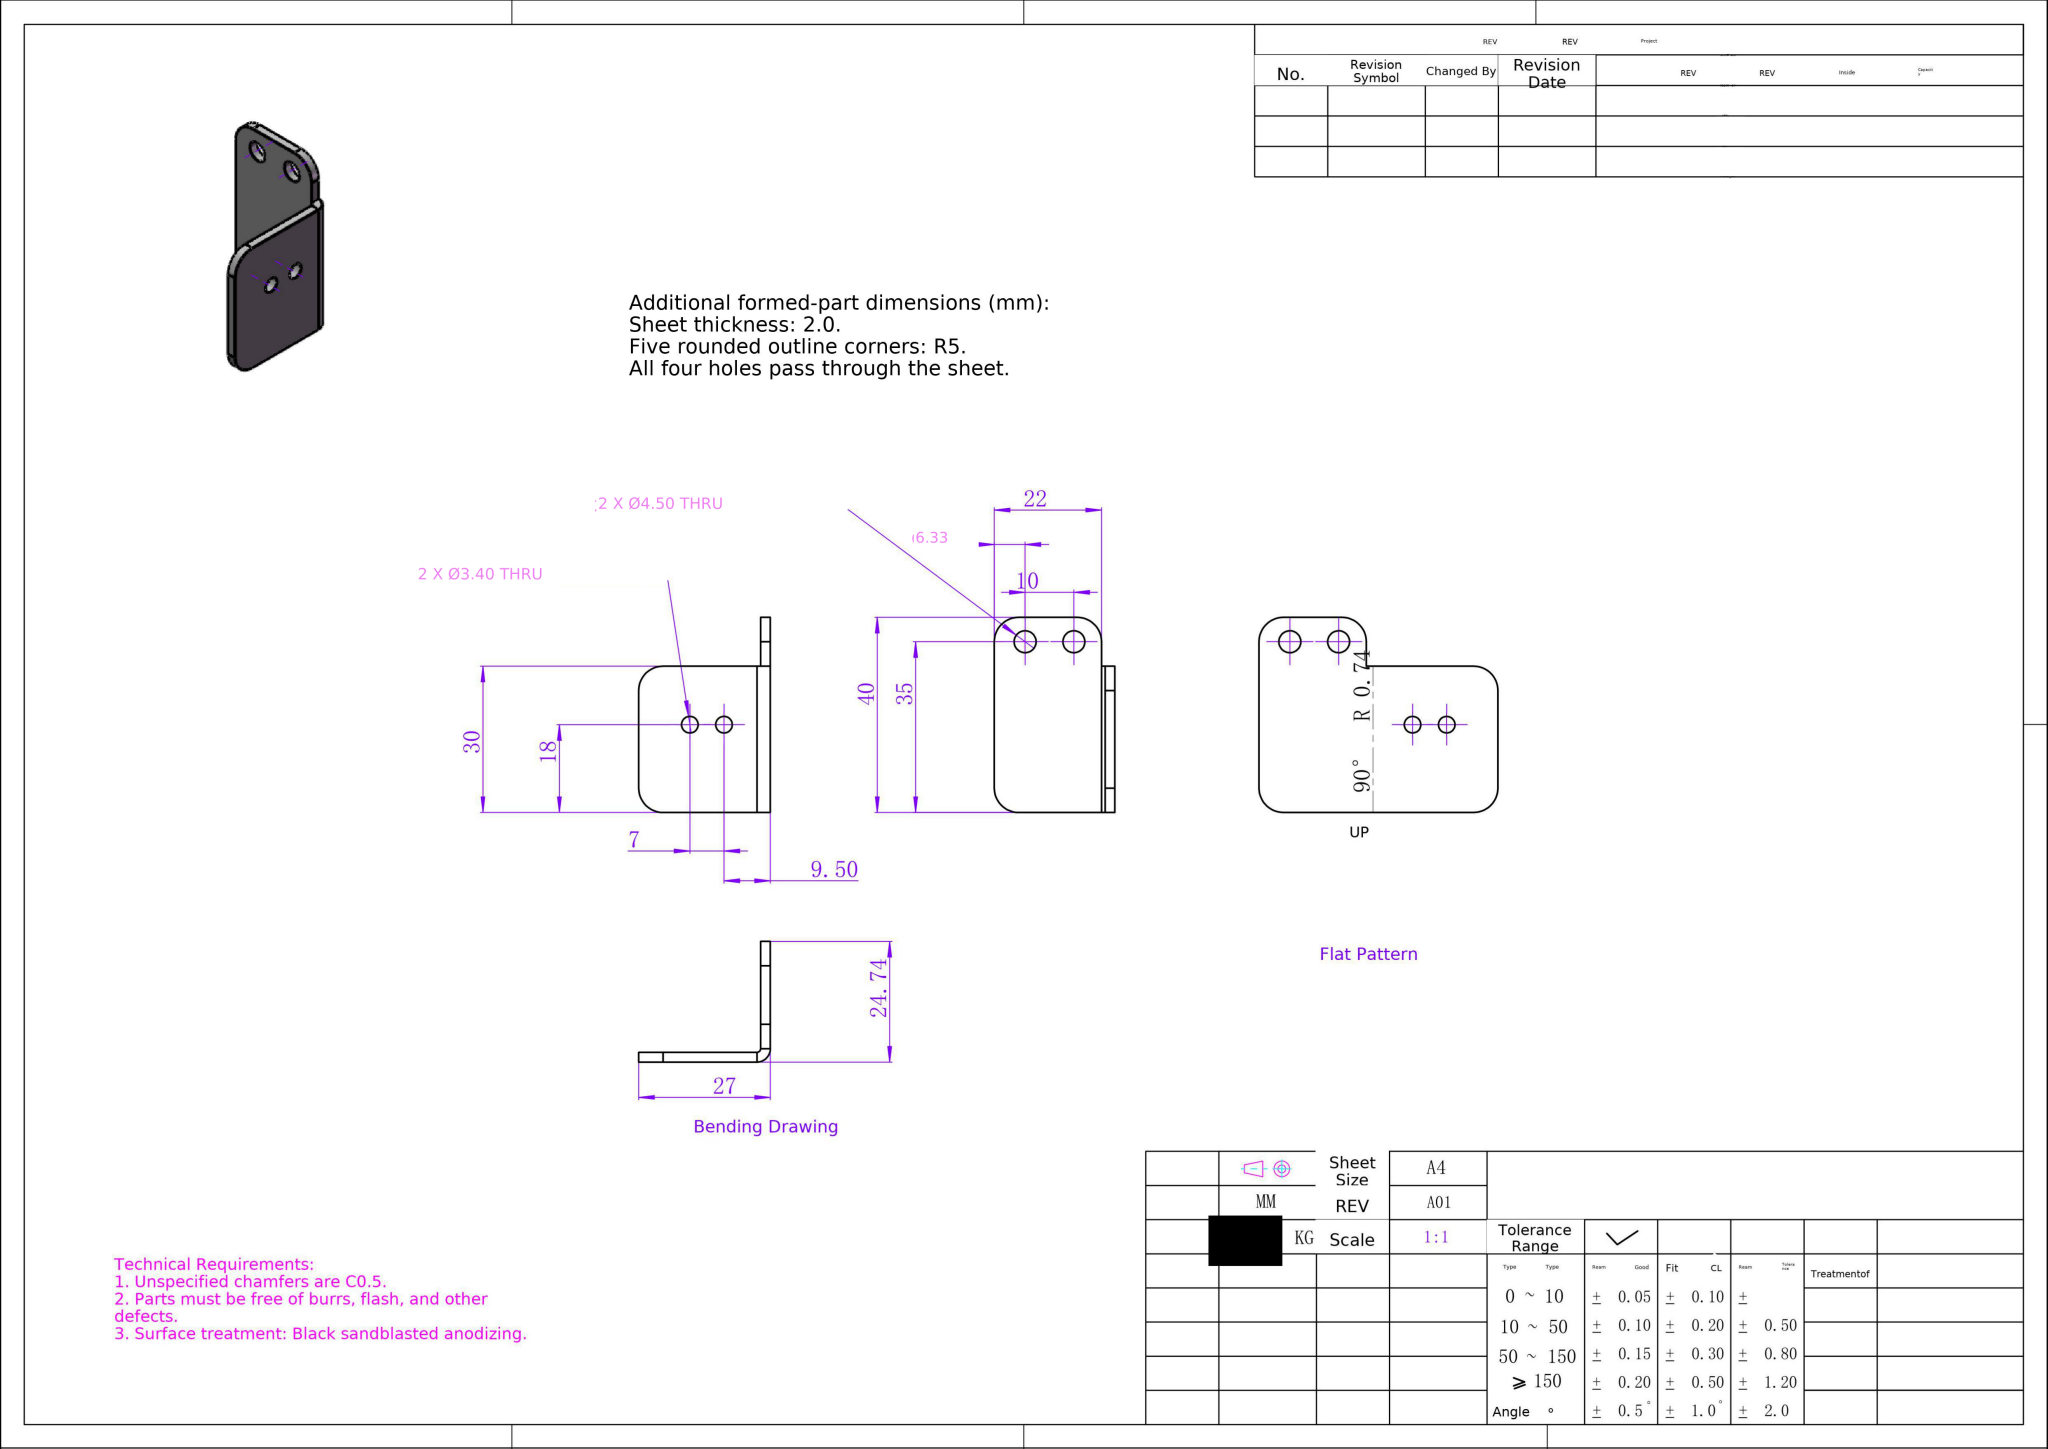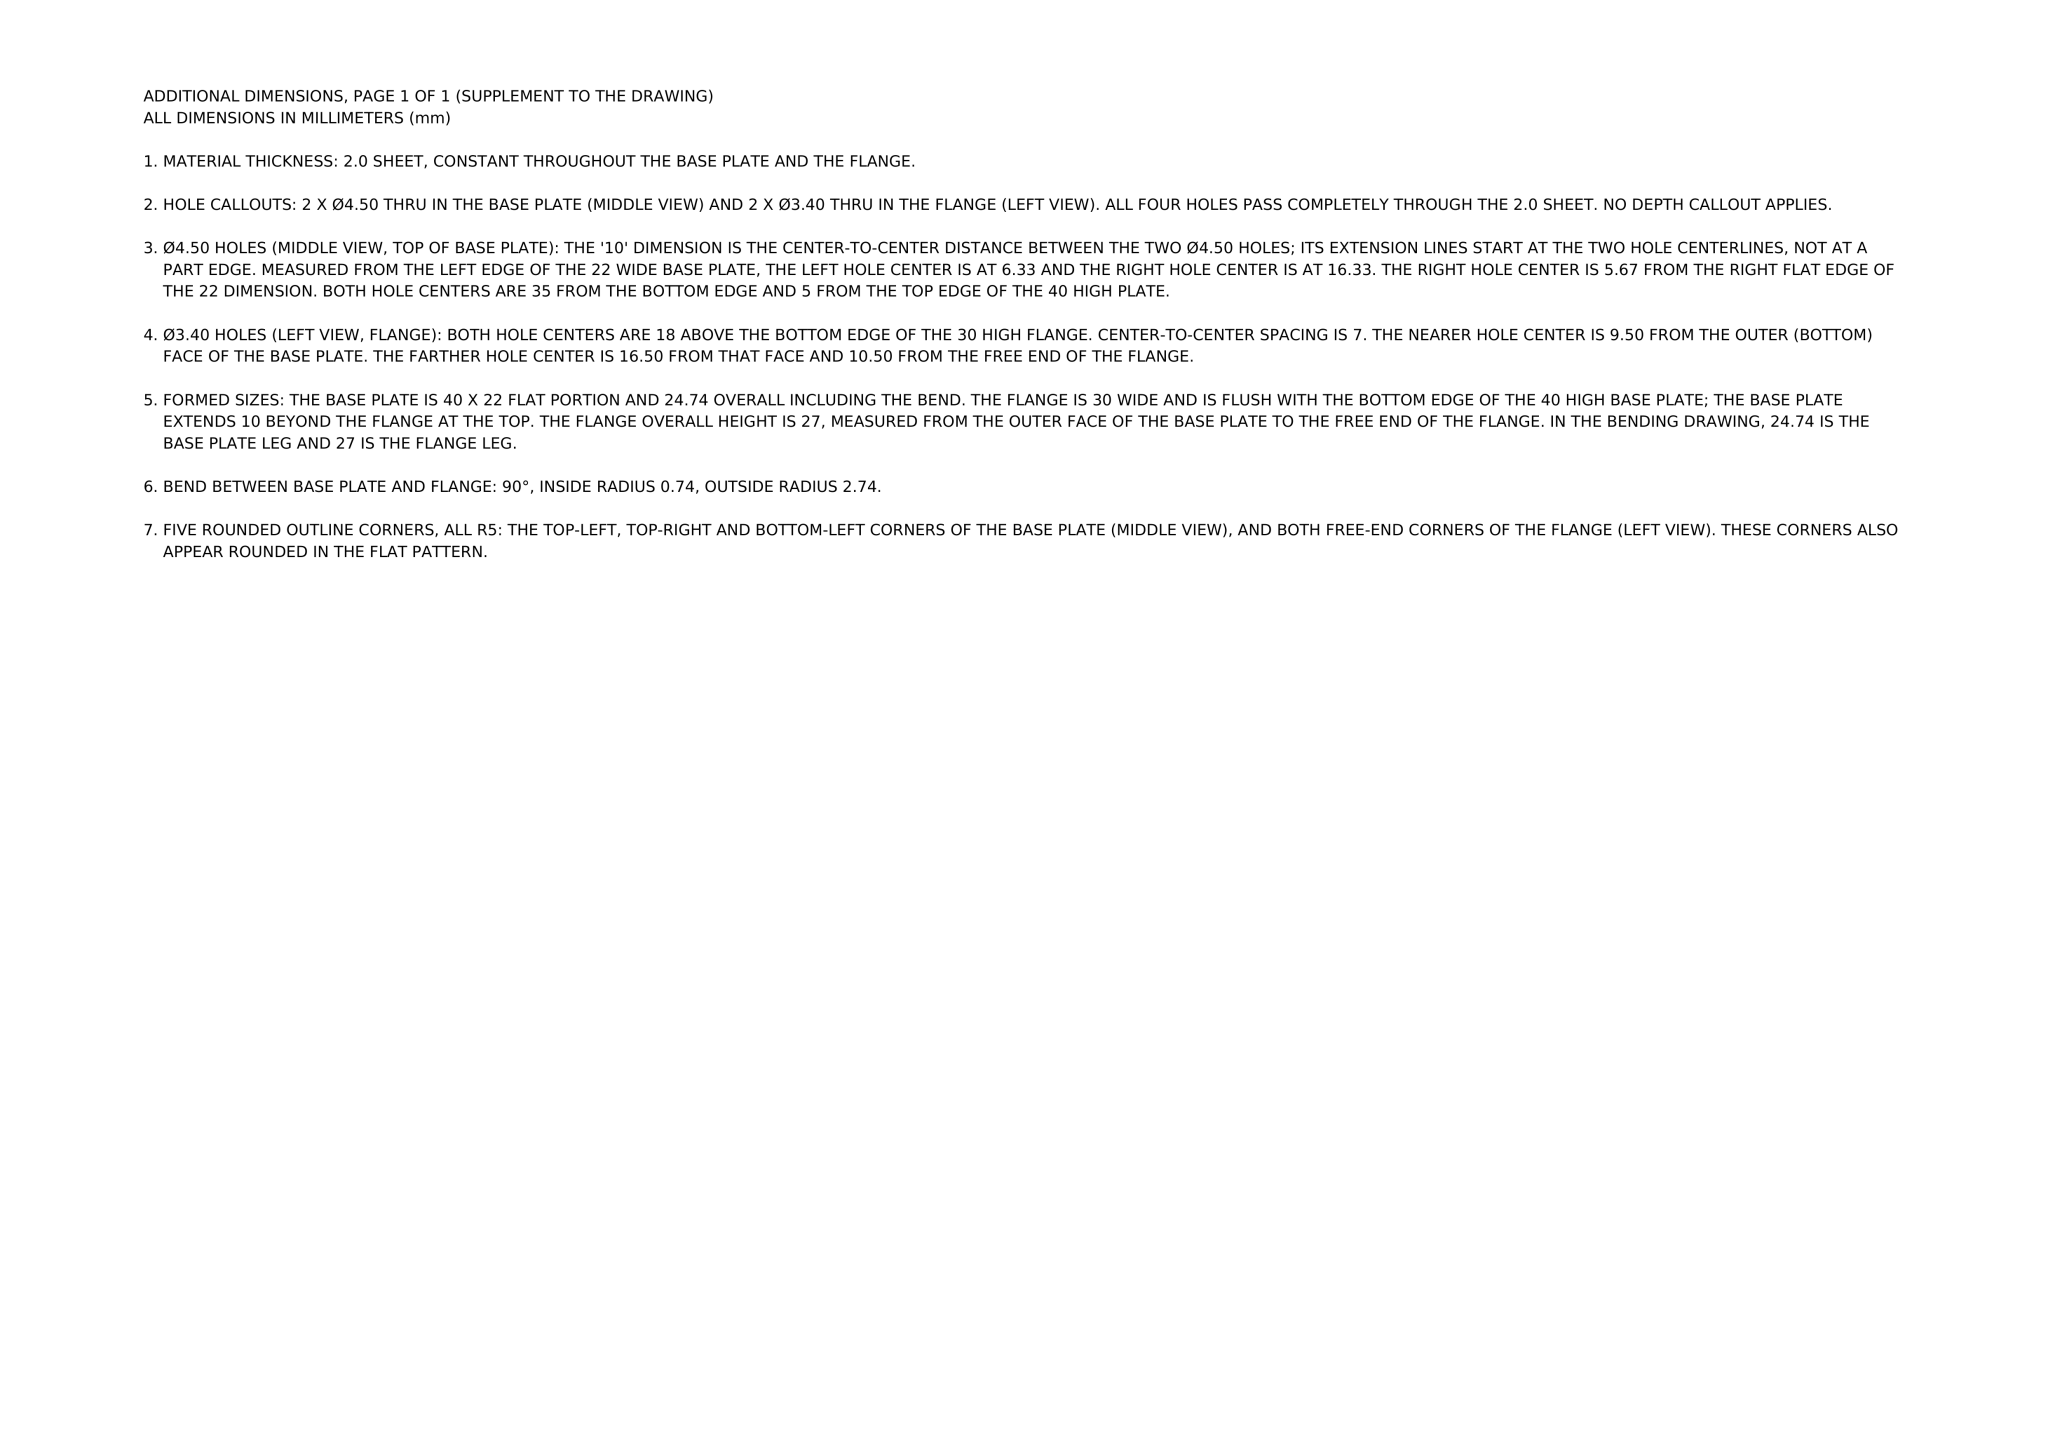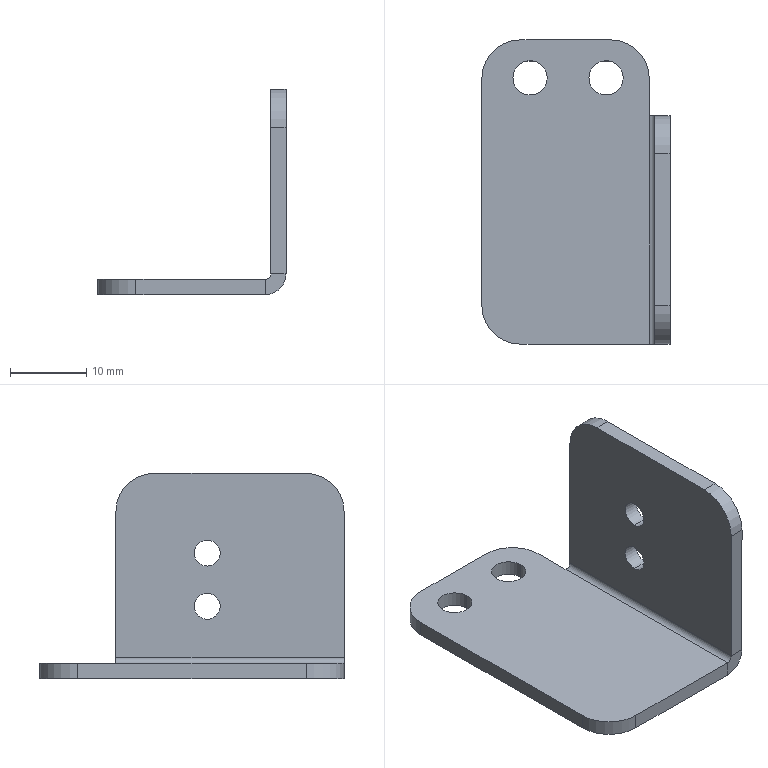Part | NX | mm | 1 solid | 28 faces | box 24.74 x 40 x 27 mm | volume 3226 mm3 | cylinder 15 | plane 13 | commonest cylinder face diameters 10 x5 3.4 x4 4.5 x4 5.473 x1 1.473 x1
STEP:
#1=COLOUR_RGB('',0.6471,0.6471,0.6471);
#2=FILL_AREA_STYLE_COLOUR('',#1);
#3=FILL_AREA_STYLE('',(#2));
#4=SURFACE_STYLE_FILL_AREA(#3);
#5=SURFACE_SIDE_STYLE('',(#4));
#6=SURFACE_STYLE_USAGE(.BOTH.,#5);
#7=PRESENTATION_STYLE_ASSIGNMENT((#6));
#8=CARTESIAN_POINT('',(46.729,-192.154,16.2));
#9=VERTEX_POINT('',#8);
#10=CARTESIAN_POINT('',(46.729,-192.154,12.8));
#11=VERTEX_POINT('',#10);
#12=CARTESIAN_POINT('',(46.729,-192.154,14.5));
#13=DIRECTION('',(1.,0.,-0.));
#14=DIRECTION('',(-0.,0.,-1.));
#15=AXIS2_PLACEMENT_3D('',#12,#13,#14);
#16=CIRCLE('',#15,1.7);
#17=EDGE_CURVE('',#9,#11,#16,.T.);
#18=ORIENTED_EDGE('',*,*,#17,.F.);
#19=CARTESIAN_POINT('',(48.729,-192.154,16.2));
#20=VERTEX_POINT('',#19);
#21=CARTESIAN_POINT('',(48.729,-192.154,16.2));
#22=DIRECTION('',(1.,0.,-0.));
#23=VECTOR('',#22,1000.);
#24=LINE('',#21,#23);
#25=EDGE_CURVE('',#9,#20,#24,.T.);
#26=ORIENTED_EDGE('',*,*,#25,.T.);
#27=CARTESIAN_POINT('',(48.729,-192.154,12.8));
#28=VERTEX_POINT('',#27);
#29=CARTESIAN_POINT('',(48.729,-192.154,14.5));
#30=DIRECTION('',(1.,0.,-0.));
#31=DIRECTION('',(-0.,0.,-1.));
#32=AXIS2_PLACEMENT_3D('',#29,#30,#31);
#33=CIRCLE('',#32,1.7);
#34=EDGE_CURVE('',#20,#28,#33,.T.);
#35=ORIENTED_EDGE('',*,*,#34,.T.);
#36=CARTESIAN_POINT('',(48.729,-192.154,12.8));
#37=DIRECTION('',(1.,0.,-0.));
#38=VECTOR('',#37,1000.);
#39=LINE('',#36,#38);
#40=EDGE_CURVE('',#11,#28,#39,.T.);
#41=ORIENTED_EDGE('',*,*,#40,.F.);
#42=EDGE_LOOP('',(#18,#26,#35,#41));
#43=FACE_OUTER_BOUND('',#42,.T.);
#44=CARTESIAN_POINT('',(48.729,-192.154,14.5));
#45=DIRECTION('',(1.,0.,-0.));
#46=DIRECTION('',(-0.,0.,-1.));
#47=AXIS2_PLACEMENT_3D('',#44,#45,#46);
#48=CYLINDRICAL_SURFACE('',#47,1.7);
#49=ADVANCED_FACE('',(#43),#48,.F.);
#50=CARTESIAN_POINT('',(46.729,-192.154,9.2));
#51=VERTEX_POINT('',#50);
#52=CARTESIAN_POINT('',(46.729,-192.154,5.8));
#53=VERTEX_POINT('',#52);
#54=CARTESIAN_POINT('',(46.729,-192.154,7.5));
#55=DIRECTION('',(1.,0.,-0.));
#56=DIRECTION('',(-0.,0.,-1.));
#57=AXIS2_PLACEMENT_3D('',#54,#55,#56);
#58=CIRCLE('',#57,1.7);
#59=EDGE_CURVE('',#51,#53,#58,.T.);
#60=ORIENTED_EDGE('',*,*,#59,.F.);
#61=CARTESIAN_POINT('',(48.729,-192.154,9.2));
#62=VERTEX_POINT('',#61);
#63=CARTESIAN_POINT('',(48.729,-192.154,9.2));
#64=DIRECTION('',(1.,0.,-0.));
#65=VECTOR('',#64,1000.);
#66=LINE('',#63,#65);
#67=EDGE_CURVE('',#51,#62,#66,.T.);
#68=ORIENTED_EDGE('',*,*,#67,.T.);
#69=CARTESIAN_POINT('',(48.729,-192.154,5.8));
#70=VERTEX_POINT('',#69);
#71=CARTESIAN_POINT('',(48.729,-192.154,7.5));
#72=DIRECTION('',(1.,0.,-0.));
#73=DIRECTION('',(-0.,0.,-1.));
#74=AXIS2_PLACEMENT_3D('',#71,#72,#73);
#75=CIRCLE('',#74,1.7);
#76=EDGE_CURVE('',#62,#70,#75,.T.);
#77=ORIENTED_EDGE('',*,*,#76,.T.);
#78=CARTESIAN_POINT('',(48.729,-192.154,5.8));
#79=DIRECTION('',(1.,0.,-0.));
#80=VECTOR('',#79,1000.);
#81=LINE('',#78,#80);
#82=EDGE_CURVE('',#53,#70,#81,.T.);
#83=ORIENTED_EDGE('',*,*,#82,.F.);
#84=EDGE_LOOP('',(#60,#68,#77,#83));
#85=FACE_OUTER_BOUND('',#84,.T.);
#86=CARTESIAN_POINT('',(48.729,-192.154,7.5));
#87=DIRECTION('',(1.,0.,-0.));
#88=DIRECTION('',(-0.,0.,-1.));
#89=AXIS2_PLACEMENT_3D('',#86,#87,#88);
#90=CYLINDRICAL_SURFACE('',#89,1.7);
#91=ADVANCED_FACE('',(#85),#90,.F.);
#92=CARTESIAN_POINT('',(38.067,-175.154,-2.));
#93=VERTEX_POINT('',#92);
#94=CARTESIAN_POINT('',(42.567,-175.154,-2.));
#95=VERTEX_POINT('',#94);
#96=CARTESIAN_POINT('',(40.317,-175.154,-2.));
#97=DIRECTION('',(0.,0.,1.));
#98=DIRECTION('',(1.,0.,0.));
#99=AXIS2_PLACEMENT_3D('',#96,#97,#98);
#100=CIRCLE('',#99,2.25);
#101=EDGE_CURVE('',#93,#95,#100,.T.);
#102=ORIENTED_EDGE('',*,*,#101,.F.);
#103=CARTESIAN_POINT('',(38.067,-175.154,0.));
#104=VERTEX_POINT('',#103);
#105=CARTESIAN_POINT('',(38.067,-175.154,0.));
#106=DIRECTION('',(0.,0.,1.));
#107=VECTOR('',#106,1000.);
#108=LINE('',#105,#107);
#109=EDGE_CURVE('',#93,#104,#108,.T.);
#110=ORIENTED_EDGE('',*,*,#109,.T.);
#111=CARTESIAN_POINT('',(42.567,-175.154,0.));
#112=VERTEX_POINT('',#111);
#113=CARTESIAN_POINT('',(40.317,-175.154,0.));
#114=DIRECTION('',(0.,0.,1.));
#115=DIRECTION('',(1.,0.,0.));
#116=AXIS2_PLACEMENT_3D('',#113,#114,#115);
#117=CIRCLE('',#116,2.25);
#118=EDGE_CURVE('',#104,#112,#117,.T.);
#119=ORIENTED_EDGE('',*,*,#118,.T.);
#120=CARTESIAN_POINT('',(42.567,-175.154,0.));
#121=DIRECTION('',(0.,0.,1.));
#122=VECTOR('',#121,1000.);
#123=LINE('',#120,#122);
#124=EDGE_CURVE('',#95,#112,#123,.T.);
#125=ORIENTED_EDGE('',*,*,#124,.F.);
#126=EDGE_LOOP('',(#102,#110,#119,#125));
#127=FACE_OUTER_BOUND('',#126,.T.);
#128=CARTESIAN_POINT('',(40.317,-175.154,0.));
#129=DIRECTION('',(0.,0.,1.));
#130=DIRECTION('',(1.,0.,0.));
#131=AXIS2_PLACEMENT_3D('',#128,#129,#130);
#132=CYLINDRICAL_SURFACE('',#131,2.25);
#133=ADVANCED_FACE('',(#127),#132,.F.);
#134=CARTESIAN_POINT('',(28.067,-175.154,-2.));
#135=VERTEX_POINT('',#134);
#136=CARTESIAN_POINT('',(32.567,-175.154,-2.));
#137=VERTEX_POINT('',#136);
#138=CARTESIAN_POINT('',(30.317,-175.154,-2.));
#139=DIRECTION('',(0.,0.,1.));
#140=DIRECTION('',(1.,0.,0.));
#141=AXIS2_PLACEMENT_3D('',#138,#139,#140);
#142=CIRCLE('',#141,2.25);
#143=EDGE_CURVE('',#135,#137,#142,.T.);
#144=ORIENTED_EDGE('',*,*,#143,.F.);
#145=CARTESIAN_POINT('',(28.067,-175.154,0.));
#146=VERTEX_POINT('',#145);
#147=CARTESIAN_POINT('',(28.067,-175.154,0.));
#148=DIRECTION('',(0.,0.,1.));
#149=VECTOR('',#148,1000.);
#150=LINE('',#147,#149);
#151=EDGE_CURVE('',#135,#146,#150,.T.);
#152=ORIENTED_EDGE('',*,*,#151,.T.);
#153=CARTESIAN_POINT('',(32.567,-175.154,0.));
#154=VERTEX_POINT('',#153);
#155=CARTESIAN_POINT('',(30.317,-175.154,0.));
#156=DIRECTION('',(0.,0.,1.));
#157=DIRECTION('',(1.,0.,0.));
#158=AXIS2_PLACEMENT_3D('',#155,#156,#157);
#159=CIRCLE('',#158,2.25);
#160=EDGE_CURVE('',#146,#154,#159,.T.);
#161=ORIENTED_EDGE('',*,*,#160,.T.);
#162=CARTESIAN_POINT('',(32.567,-175.154,0.));
#163=DIRECTION('',(0.,0.,1.));
#164=VECTOR('',#163,1000.);
#165=LINE('',#162,#164);
#166=EDGE_CURVE('',#137,#154,#165,.T.);
#167=ORIENTED_EDGE('',*,*,#166,.F.);
#168=EDGE_LOOP('',(#144,#152,#161,#167));
#169=FACE_OUTER_BOUND('',#168,.T.);
#170=CARTESIAN_POINT('',(30.317,-175.154,0.));
#171=DIRECTION('',(0.,0.,1.));
#172=DIRECTION('',(1.,0.,0.));
#173=AXIS2_PLACEMENT_3D('',#170,#171,#172);
#174=CYLINDRICAL_SURFACE('',#173,2.25);
#175=ADVANCED_FACE('',(#169),#174,.F.);
#176=CARTESIAN_POINT('',(45.993,-180.154,-2.));
#177=VERTEX_POINT('',#176);
#178=CARTESIAN_POINT('',(45.993,-175.154,-2.));
#179=VERTEX_POINT('',#178);
#180=CARTESIAN_POINT('',(45.993,-170.154,-2.));
#181=DIRECTION('',(-0.,1.,0.));
#182=VECTOR('',#181,1000.);
#183=LINE('',#180,#182);
#184=EDGE_CURVE('',#177,#179,#183,.T.);
#185=ORIENTED_EDGE('',*,*,#184,.T.);
#186=CARTESIAN_POINT('',(45.993,-175.154,0.));
#187=VERTEX_POINT('',#186);
#188=CARTESIAN_POINT('',(45.993,-175.154,-2.));
#189=DIRECTION('',(0.,0.,1.));
#190=VECTOR('',#189,1000.);
#191=LINE('',#188,#190);
#192=EDGE_CURVE('',#179,#187,#191,.T.);
#193=ORIENTED_EDGE('',*,*,#192,.T.);
#194=CARTESIAN_POINT('',(45.993,-180.154,0.));
#195=VERTEX_POINT('',#194);
#196=CARTESIAN_POINT('',(45.993,-170.154,0.));
#197=DIRECTION('',(-0.,1.,0.));
#198=VECTOR('',#197,1000.);
#199=LINE('',#196,#198);
#200=EDGE_CURVE('',#195,#187,#199,.T.);
#201=ORIENTED_EDGE('',*,*,#200,.F.);
#202=CARTESIAN_POINT('',(45.993,-180.154,0.));
#203=DIRECTION('',(0.,0.,-1.));
#204=VECTOR('',#203,1000.);
#205=LINE('',#202,#204);
#206=EDGE_CURVE('',#195,#177,#205,.T.);
#207=ORIENTED_EDGE('',*,*,#206,.T.);
#208=EDGE_LOOP('',(#185,#193,#201,#207));
#209=FACE_OUTER_BOUND('',#208,.T.);
#210=CARTESIAN_POINT('',(45.993,-170.154,-2.));
#211=DIRECTION('',(1.,0.,0.));
#212=DIRECTION('',(-0.,1.,0.));
#213=AXIS2_PLACEMENT_3D('',#210,#211,#212);
#214=PLANE('',#213);
#215=ADVANCED_FACE('',(#209),#214,.T.);
#216=CARTESIAN_POINT('',(23.993,-175.154,0.));
#217=VERTEX_POINT('',#216);
#218=CARTESIAN_POINT('',(23.993,-205.154,0.));
#219=VERTEX_POINT('',#218);
#220=CARTESIAN_POINT('',(23.993,-170.154,0.));
#221=DIRECTION('',(0.,-1.,0.));
#222=VECTOR('',#221,1000.);
#223=LINE('',#220,#222);
#224=EDGE_CURVE('',#217,#219,#223,.T.);
#225=ORIENTED_EDGE('',*,*,#224,.F.);
#226=CARTESIAN_POINT('',(23.993,-175.154,-2.));
#227=VERTEX_POINT('',#226);
#228=CARTESIAN_POINT('',(23.993,-175.154,-2.));
#229=DIRECTION('',(0.,0.,-1.));
#230=VECTOR('',#229,1000.);
#231=LINE('',#228,#230);
#232=EDGE_CURVE('',#217,#227,#231,.T.);
#233=ORIENTED_EDGE('',*,*,#232,.T.);
#234=CARTESIAN_POINT('',(23.993,-205.154,-2.));
#235=VERTEX_POINT('',#234);
#236=CARTESIAN_POINT('',(23.993,-170.154,-2.));
#237=DIRECTION('',(0.,-1.,0.));
#238=VECTOR('',#237,1000.);
#239=LINE('',#236,#238);
#240=EDGE_CURVE('',#227,#235,#239,.T.);
#241=ORIENTED_EDGE('',*,*,#240,.T.);
#242=CARTESIAN_POINT('',(23.993,-205.154,-2.));
#243=DIRECTION('',(0.,0.,1.));
#244=VECTOR('',#243,1000.);
#245=LINE('',#242,#244);
#246=EDGE_CURVE('',#235,#219,#245,.T.);
#247=ORIENTED_EDGE('',*,*,#246,.T.);
#248=EDGE_LOOP('',(#225,#233,#241,#247));
#249=FACE_OUTER_BOUND('',#248,.T.);
#250=CARTESIAN_POINT('',(23.993,-170.154,-2.));
#251=DIRECTION('',(-1.,-0.,0.));
#252=DIRECTION('',(0.,-1.,0.));
#253=AXIS2_PLACEMENT_3D('',#250,#251,#252);
#254=PLANE('',#253);
#255=ADVANCED_FACE('',(#249),#254,.T.);
#256=CARTESIAN_POINT('',(40.993,-170.154,-2.));
#257=VERTEX_POINT('',#256);
#258=CARTESIAN_POINT('',(28.993,-170.154,-2.));
#259=VERTEX_POINT('',#258);
#260=CARTESIAN_POINT('',(23.993,-170.154,-2.));
#261=DIRECTION('',(-1.,0.,0.));
#262=VECTOR('',#261,1000.);
#263=LINE('',#260,#262);
#264=EDGE_CURVE('',#257,#259,#263,.T.);
#265=ORIENTED_EDGE('',*,*,#264,.T.);
#266=CARTESIAN_POINT('',(28.993,-170.154,0.));
#267=VERTEX_POINT('',#266);
#268=CARTESIAN_POINT('',(28.993,-170.154,-2.));
#269=DIRECTION('',(0.,0.,1.));
#270=VECTOR('',#269,1000.);
#271=LINE('',#268,#270);
#272=EDGE_CURVE('',#259,#267,#271,.T.);
#273=ORIENTED_EDGE('',*,*,#272,.T.);
#274=CARTESIAN_POINT('',(40.993,-170.154,0.));
#275=VERTEX_POINT('',#274);
#276=CARTESIAN_POINT('',(23.993,-170.154,0.));
#277=DIRECTION('',(-1.,0.,0.));
#278=VECTOR('',#277,1000.);
#279=LINE('',#276,#278);
#280=EDGE_CURVE('',#275,#267,#279,.T.);
#281=ORIENTED_EDGE('',*,*,#280,.F.);
#282=CARTESIAN_POINT('',(40.993,-170.154,-2.));
#283=DIRECTION('',(0.,0.,-1.));
#284=VECTOR('',#283,1000.);
#285=LINE('',#282,#284);
#286=EDGE_CURVE('',#275,#257,#285,.T.);
#287=ORIENTED_EDGE('',*,*,#286,.T.);
#288=EDGE_LOOP('',(#265,#273,#281,#287));
#289=FACE_OUTER_BOUND('',#288,.T.);
#290=CARTESIAN_POINT('',(23.993,-170.154,-2.));
#291=DIRECTION('',(0.,1.,0.));
#292=DIRECTION('',(0.,0.,1.));
#293=AXIS2_PLACEMENT_3D('',#290,#291,#292);
#294=PLANE('',#293);
#295=ADVANCED_FACE('',(#289),#294,.T.);
#296=CARTESIAN_POINT('',(28.993,-210.154,0.));
#297=VERTEX_POINT('',#296);
#298=CARTESIAN_POINT('',(45.993,-210.154,0.));
#299=VERTEX_POINT('',#298);
#300=CARTESIAN_POINT('',(23.993,-210.154,0.));
#301=DIRECTION('',(1.,0.,0.));
#302=VECTOR('',#301,1000.);
#303=LINE('',#300,#302);
#304=EDGE_CURVE('',#297,#299,#303,.T.);
#305=ORIENTED_EDGE('',*,*,#304,.F.);
#306=CARTESIAN_POINT('',(28.993,-210.154,-2.));
#307=VERTEX_POINT('',#306);
#308=CARTESIAN_POINT('',(28.993,-210.154,-2.));
#309=DIRECTION('',(0.,0.,-1.));
#310=VECTOR('',#309,1000.);
#311=LINE('',#308,#310);
#312=EDGE_CURVE('',#297,#307,#311,.T.);
#313=ORIENTED_EDGE('',*,*,#312,.T.);
#314=CARTESIAN_POINT('',(45.993,-210.154,-2.));
#315=VERTEX_POINT('',#314);
#316=CARTESIAN_POINT('',(23.993,-210.154,-2.));
#317=DIRECTION('',(1.,0.,0.));
#318=VECTOR('',#317,1000.);
#319=LINE('',#316,#318);
#320=EDGE_CURVE('',#307,#315,#319,.T.);
#321=ORIENTED_EDGE('',*,*,#320,.T.);
#322=CARTESIAN_POINT('',(45.993,-210.154,-2.));
#323=DIRECTION('',(0.,0.,1.));
#324=VECTOR('',#323,1000.);
#325=LINE('',#322,#324);
#326=EDGE_CURVE('',#315,#299,#325,.T.);
#327=ORIENTED_EDGE('',*,*,#326,.T.);
#328=EDGE_LOOP('',(#305,#313,#321,#327));
#329=FACE_OUTER_BOUND('',#328,.T.);
#330=CARTESIAN_POINT('',(23.993,-210.154,-2.));
#331=DIRECTION('',(0.,-1.,0.));
#332=DIRECTION('',(0.,0.,-1.));
#333=AXIS2_PLACEMENT_3D('',#330,#331,#332);
#334=PLANE('',#333);
#335=ADVANCED_FACE('',(#329),#334,.T.);
#336=CARTESIAN_POINT('',(40.317,-175.154,-2.));
#337=DIRECTION('',(0.,0.,1.));
#338=DIRECTION('',(1.,0.,0.));
#339=AXIS2_PLACEMENT_3D('',#336,#337,#338);
#340=CIRCLE('',#339,2.25);
#341=EDGE_CURVE('',#95,#93,#340,.T.);
#342=ORIENTED_EDGE('',*,*,#341,.T.);
#343=ORIENTED_EDGE('',*,*,#101,.T.);
#344=EDGE_LOOP('',(#342,#343));
#345=FACE_BOUND('',#344,.T.);
#346=CARTESIAN_POINT('',(30.317,-175.154,-2.));
#347=DIRECTION('',(0.,0.,1.));
#348=DIRECTION('',(1.,0.,0.));
#349=AXIS2_PLACEMENT_3D('',#346,#347,#348);
#350=CIRCLE('',#349,2.25);
#351=EDGE_CURVE('',#137,#135,#350,.T.);
#352=ORIENTED_EDGE('',*,*,#351,.T.);
#353=ORIENTED_EDGE('',*,*,#143,.T.);
#354=EDGE_LOOP('',(#352,#353));
#355=FACE_BOUND('',#354,.T.);
#356=ORIENTED_EDGE('',*,*,#240,.F.);
#357=CARTESIAN_POINT('',(28.993,-175.154,-2.));
#358=DIRECTION('',(0.,0.,-1.));
#359=DIRECTION('',(1.,0.,0.));
#360=AXIS2_PLACEMENT_3D('',#357,#358,#359);
#361=CIRCLE('',#360,5.);
#362=EDGE_CURVE('',#227,#259,#361,.T.);
#363=ORIENTED_EDGE('',*,*,#362,.T.);
#364=ORIENTED_EDGE('',*,*,#264,.F.);
#365=CARTESIAN_POINT('',(40.993,-175.154,-2.));
#366=DIRECTION('',(0.,0.,-1.));
#367=DIRECTION('',(1.,0.,0.));
#368=AXIS2_PLACEMENT_3D('',#365,#366,#367);
#369=CIRCLE('',#368,5.);
#370=EDGE_CURVE('',#257,#179,#369,.T.);
#371=ORIENTED_EDGE('',*,*,#370,.T.);
#372=ORIENTED_EDGE('',*,*,#184,.F.);
#373=CARTESIAN_POINT('',(45.993,-170.154,-2.));
#374=DIRECTION('',(-0.,1.,0.));
#375=VECTOR('',#374,1000.);
#376=LINE('',#373,#375);
#377=EDGE_CURVE('',#315,#177,#376,.T.);
#378=ORIENTED_EDGE('',*,*,#377,.F.);
#379=ORIENTED_EDGE('',*,*,#320,.F.);
#380=CARTESIAN_POINT('',(28.993,-205.154,-2.));
#381=DIRECTION('',(0.,0.,-1.));
#382=DIRECTION('',(1.,0.,0.));
#383=AXIS2_PLACEMENT_3D('',#380,#381,#382);
#384=CIRCLE('',#383,5.);
#385=EDGE_CURVE('',#307,#235,#384,.T.);
#386=ORIENTED_EDGE('',*,*,#385,.T.);
#387=EDGE_LOOP('',(#356,#363,#364,#371,#372,#378,#379,#386));
#388=FACE_OUTER_BOUND('',#387,.T.);
#389=CARTESIAN_POINT('',(0.,0.,-2.));
#390=DIRECTION('',(0.,0.,1.));
#391=DIRECTION('',(1.,0.,0.));
#392=AXIS2_PLACEMENT_3D('',#389,#390,#391);
#393=PLANE('',#392);
#394=ADVANCED_FACE('',(#345,#355,#388),#393,.F.);
#395=CARTESIAN_POINT('',(40.317,-175.154,0.));
#396=DIRECTION('',(0.,0.,1.));
#397=DIRECTION('',(1.,0.,0.));
#398=AXIS2_PLACEMENT_3D('',#395,#396,#397);
#399=CIRCLE('',#398,2.25);
#400=EDGE_CURVE('',#112,#104,#399,.T.);
#401=ORIENTED_EDGE('',*,*,#400,.F.);
#402=ORIENTED_EDGE('',*,*,#118,.F.);
#403=EDGE_LOOP('',(#401,#402));
#404=FACE_BOUND('',#403,.T.);
#405=CARTESIAN_POINT('',(30.317,-175.154,0.));
#406=DIRECTION('',(0.,0.,1.));
#407=DIRECTION('',(1.,0.,0.));
#408=AXIS2_PLACEMENT_3D('',#405,#406,#407);
#409=CIRCLE('',#408,2.25);
#410=EDGE_CURVE('',#154,#146,#409,.T.);
#411=ORIENTED_EDGE('',*,*,#410,.F.);
#412=ORIENTED_EDGE('',*,*,#160,.F.);
#413=EDGE_LOOP('',(#411,#412));
#414=FACE_BOUND('',#413,.T.);
#415=ORIENTED_EDGE('',*,*,#280,.T.);
#416=CARTESIAN_POINT('',(28.993,-175.154,0.));
#417=DIRECTION('',(0.,0.,1.));
#418=DIRECTION('',(1.,0.,0.));
#419=AXIS2_PLACEMENT_3D('',#416,#417,#418);
#420=CIRCLE('',#419,5.);
#421=EDGE_CURVE('',#267,#217,#420,.T.);
#422=ORIENTED_EDGE('',*,*,#421,.T.);
#423=ORIENTED_EDGE('',*,*,#224,.T.);
#424=CARTESIAN_POINT('',(28.993,-205.154,0.));
#425=DIRECTION('',(0.,0.,1.));
#426=DIRECTION('',(1.,0.,0.));
#427=AXIS2_PLACEMENT_3D('',#424,#425,#426);
#428=CIRCLE('',#427,5.);
#429=EDGE_CURVE('',#219,#297,#428,.T.);
#430=ORIENTED_EDGE('',*,*,#429,.T.);
#431=ORIENTED_EDGE('',*,*,#304,.T.);
#432=CARTESIAN_POINT('',(45.993,-170.154,0.));
#433=DIRECTION('',(-0.,1.,0.));
#434=VECTOR('',#433,1000.);
#435=LINE('',#432,#434);
#436=EDGE_CURVE('',#299,#195,#435,.T.);
#437=ORIENTED_EDGE('',*,*,#436,.T.);
#438=ORIENTED_EDGE('',*,*,#200,.T.);
#439=CARTESIAN_POINT('',(40.993,-175.154,0.));
#440=DIRECTION('',(0.,0.,1.));
#441=DIRECTION('',(1.,0.,0.));
#442=AXIS2_PLACEMENT_3D('',#439,#440,#441);
#443=CIRCLE('',#442,5.);
#444=EDGE_CURVE('',#187,#275,#443,.T.);
#445=ORIENTED_EDGE('',*,*,#444,.T.);
#446=EDGE_LOOP('',(#415,#422,#423,#430,#431,#437,#438,#445));
#447=FACE_OUTER_BOUND('',#446,.T.);
#448=CARTESIAN_POINT('',(0.,0.,0.));
#449=DIRECTION('',(0.,0.,1.));
#450=DIRECTION('',(1.,0.,0.));
#451=AXIS2_PLACEMENT_3D('',#448,#449,#450);
#452=PLANE('',#451);
#453=ADVANCED_FACE('',(#404,#414,#447),#452,.T.);
#454=CARTESIAN_POINT('',(46.729,-210.154,0.7366));
#455=VERTEX_POINT('',#454);
#456=CARTESIAN_POINT('',(48.729,-210.154,0.7366));
#457=VERTEX_POINT('',#456);
#458=CARTESIAN_POINT('',(48.729,-210.154,0.7366));
#459=DIRECTION('',(1.,0.,-0.));
#460=VECTOR('',#459,1000.);
#461=LINE('',#458,#460);
#462=EDGE_CURVE('',#455,#457,#461,.T.);
#463=ORIENTED_EDGE('',*,*,#462,.F.);
#464=CARTESIAN_POINT('',(45.993,-210.154,0.7366));
#465=DIRECTION('',(0.,-1.,0.));
#466=DIRECTION('',(0.,0.,1.));
#467=AXIS2_PLACEMENT_3D('',#464,#465,#466);
#468=CIRCLE('',#467,0.7366);
#469=EDGE_CURVE('',#299,#455,#468,.T.);
#470=ORIENTED_EDGE('',*,*,#469,.F.);
#471=ORIENTED_EDGE('',*,*,#326,.F.);
#472=CARTESIAN_POINT('',(45.993,-210.154,0.7366));
#473=DIRECTION('',(0.,-1.,0.));
#474=DIRECTION('',(0.,0.,1.));
#475=AXIS2_PLACEMENT_3D('',#472,#473,#474);
#476=CIRCLE('',#475,2.737);
#477=EDGE_CURVE('',#315,#457,#476,.T.);
#478=ORIENTED_EDGE('',*,*,#477,.T.);
#479=EDGE_LOOP('',(#463,#470,#471,#478));
#480=FACE_OUTER_BOUND('',#479,.T.);
#481=CARTESIAN_POINT('',(45.993,-210.154,0.7366));
#482=DIRECTION('',(0.,-1.,0.));
#483=DIRECTION('',(0.,0.,-1.));
#484=AXIS2_PLACEMENT_3D('',#481,#482,#483);
#485=PLANE('',#484);
#486=ADVANCED_FACE('',(#480),#485,.T.);
#487=CARTESIAN_POINT('',(46.729,-180.154,0.7366));
#488=VERTEX_POINT('',#487);
#489=CARTESIAN_POINT('',(45.993,-180.154,0.7366));
#490=DIRECTION('',(0.,1.,0.));
#491=DIRECTION('',(0.,0.,1.));
#492=AXIS2_PLACEMENT_3D('',#489,#490,#491);
#493=CIRCLE('',#492,0.7366);
#494=EDGE_CURVE('',#488,#195,#493,.T.);
#495=ORIENTED_EDGE('',*,*,#494,.F.);
#496=CARTESIAN_POINT('',(48.729,-180.154,0.7366));
#497=VERTEX_POINT('',#496);
#498=CARTESIAN_POINT('',(46.729,-180.154,0.7366));
#499=DIRECTION('',(1.,0.,-0.));
#500=VECTOR('',#499,1000.);
#501=LINE('',#498,#500);
#502=EDGE_CURVE('',#488,#497,#501,.T.);
#503=ORIENTED_EDGE('',*,*,#502,.T.);
#504=CARTESIAN_POINT('',(45.993,-180.154,0.7366));
#505=DIRECTION('',(0.,1.,0.));
#506=DIRECTION('',(0.,0.,1.));
#507=AXIS2_PLACEMENT_3D('',#504,#505,#506);
#508=CIRCLE('',#507,2.737);
#509=EDGE_CURVE('',#497,#177,#508,.T.);
#510=ORIENTED_EDGE('',*,*,#509,.T.);
#511=ORIENTED_EDGE('',*,*,#206,.F.);
#512=EDGE_LOOP('',(#495,#503,#510,#511));
#513=FACE_OUTER_BOUND('',#512,.T.);
#514=CARTESIAN_POINT('',(45.993,-180.154,0.7366));
#515=DIRECTION('',(0.,-1.,0.));
#516=DIRECTION('',(0.,0.,-1.));
#517=AXIS2_PLACEMENT_3D('',#514,#515,#516);
#518=PLANE('',#517);
#519=ADVANCED_FACE('',(#513),#518,.F.);
#520=ORIENTED_EDGE('',*,*,#377,.T.);
#521=ORIENTED_EDGE('',*,*,#509,.F.);
#522=CARTESIAN_POINT('',(48.729,0.,0.7366));
#523=DIRECTION('',(-0.,1.,0.));
#524=VECTOR('',#523,1000.);
#525=LINE('',#522,#524);
#526=EDGE_CURVE('',#457,#497,#525,.T.);
#527=ORIENTED_EDGE('',*,*,#526,.F.);
#528=ORIENTED_EDGE('',*,*,#477,.F.);
#529=EDGE_LOOP('',(#520,#521,#527,#528));
#530=FACE_OUTER_BOUND('',#529,.T.);
#531=CARTESIAN_POINT('',(45.993,-180.154,0.7366));
#532=DIRECTION('',(0.,1.,0.));
#533=DIRECTION('',(1.,0.,-0.));
#534=AXIS2_PLACEMENT_3D('',#531,#532,#533);
#535=CYLINDRICAL_SURFACE('',#534,2.737);
#536=ADVANCED_FACE('',(#530),#535,.T.);
#537=ORIENTED_EDGE('',*,*,#436,.F.);
#538=ORIENTED_EDGE('',*,*,#469,.T.);
#539=CARTESIAN_POINT('',(46.729,-210.154,0.7366));
#540=DIRECTION('',(-0.,1.,0.));
#541=VECTOR('',#540,1000.);
#542=LINE('',#539,#541);
#543=EDGE_CURVE('',#455,#488,#542,.T.);
#544=ORIENTED_EDGE('',*,*,#543,.T.);
#545=ORIENTED_EDGE('',*,*,#494,.T.);
#546=EDGE_LOOP('',(#537,#538,#544,#545));
#547=FACE_OUTER_BOUND('',#546,.T.);
#548=CARTESIAN_POINT('',(45.993,-180.154,0.7366));
#549=DIRECTION('',(0.,1.,0.));
#550=DIRECTION('',(1.,0.,-0.));
#551=AXIS2_PLACEMENT_3D('',#548,#549,#550);
#552=CYLINDRICAL_SURFACE('',#551,0.7366);
#553=ADVANCED_FACE('',(#547),#552,.F.);
#554=CARTESIAN_POINT('',(46.729,-180.154,20.));
#555=VERTEX_POINT('',#554);
#556=CARTESIAN_POINT('',(46.729,-180.154,25.));
#557=DIRECTION('',(0.,0.,1.));
#558=VECTOR('',#557,1000.);
#559=LINE('',#556,#558);
#560=EDGE_CURVE('',#488,#555,#559,.T.);
#561=ORIENTED_EDGE('',*,*,#560,.T.);
#562=CARTESIAN_POINT('',(48.729,-180.154,20.));
#563=VERTEX_POINT('',#562);
#564=CARTESIAN_POINT('',(48.729,-180.154,20.));
#565=DIRECTION('',(1.,0.,-0.));
#566=VECTOR('',#565,1000.);
#567=LINE('',#564,#566);
#568=EDGE_CURVE('',#555,#563,#567,.T.);
#569=ORIENTED_EDGE('',*,*,#568,.T.);
#570=CARTESIAN_POINT('',(48.729,-180.154,0.));
#571=DIRECTION('',(0.,0.,1.));
#572=VECTOR('',#571,1000.);
#573=LINE('',#570,#572);
#574=EDGE_CURVE('',#497,#563,#573,.T.);
#575=ORIENTED_EDGE('',*,*,#574,.F.);
#576=ORIENTED_EDGE('',*,*,#502,.F.);
#577=EDGE_LOOP('',(#561,#569,#575,#576));
#578=FACE_OUTER_BOUND('',#577,.T.);
#579=CARTESIAN_POINT('',(48.729,-180.154,25.));
#580=DIRECTION('',(0.,-1.,0.));
#581=DIRECTION('',(0.,-0.,-1.));
#582=AXIS2_PLACEMENT_3D('',#579,#580,#581);
#583=PLANE('',#582);
#584=ADVANCED_FACE('',(#578),#583,.F.);
#585=CARTESIAN_POINT('',(48.729,-210.154,20.));
#586=VERTEX_POINT('',#585);
#587=CARTESIAN_POINT('',(48.729,-210.154,-0.));
#588=DIRECTION('',(-0.,0.,-1.));
#589=VECTOR('',#588,1000.);
#590=LINE('',#587,#589);
#591=EDGE_CURVE('',#586,#457,#590,.T.);
#592=ORIENTED_EDGE('',*,*,#591,.F.);
#593=CARTESIAN_POINT('',(46.729,-210.154,20.));
#594=VERTEX_POINT('',#593);
#595=CARTESIAN_POINT('',(48.729,-210.154,20.));
#596=DIRECTION('',(-1.,-0.,0.));
#597=VECTOR('',#596,1000.);
#598=LINE('',#595,#597);
#599=EDGE_CURVE('',#586,#594,#598,.T.);
#600=ORIENTED_EDGE('',*,*,#599,.T.);
#601=CARTESIAN_POINT('',(46.729,-210.154,-0.));
#602=DIRECTION('',(-0.,0.,-1.));
#603=VECTOR('',#602,1000.);
#604=LINE('',#601,#603);
#605=EDGE_CURVE('',#594,#455,#604,.T.);
#606=ORIENTED_EDGE('',*,*,#605,.T.);
#607=ORIENTED_EDGE('',*,*,#462,.T.);
#608=EDGE_LOOP('',(#592,#600,#606,#607));
#609=FACE_OUTER_BOUND('',#608,.T.);
#610=CARTESIAN_POINT('',(48.729,-210.154,-0.));
#611=DIRECTION('',(-0.,1.,0.));
#612=DIRECTION('',(-1.,-0.,0.));
#613=AXIS2_PLACEMENT_3D('',#610,#611,#612);
#614=PLANE('',#613);
#615=ADVANCED_FACE('',(#609),#614,.F.);
#616=CARTESIAN_POINT('',(48.729,-192.154,14.5));
#617=DIRECTION('',(1.,0.,-0.));
#618=DIRECTION('',(-0.,0.,-1.));
#619=AXIS2_PLACEMENT_3D('',#616,#617,#618);
#620=CIRCLE('',#619,1.7);
#621=EDGE_CURVE('',#28,#20,#620,.T.);
#622=ORIENTED_EDGE('',*,*,#621,.F.);
#623=ORIENTED_EDGE('',*,*,#34,.F.);
#624=EDGE_LOOP('',(#622,#623));
#625=FACE_BOUND('',#624,.T.);
#626=CARTESIAN_POINT('',(48.729,-192.154,7.5));
#627=DIRECTION('',(1.,0.,-0.));
#628=DIRECTION('',(-0.,0.,-1.));
#629=AXIS2_PLACEMENT_3D('',#626,#627,#628);
#630=CIRCLE('',#629,1.7);
#631=EDGE_CURVE('',#70,#62,#630,.T.);
#632=ORIENTED_EDGE('',*,*,#631,.F.);
#633=ORIENTED_EDGE('',*,*,#76,.F.);
#634=EDGE_LOOP('',(#632,#633));
#635=FACE_BOUND('',#634,.T.);
#636=CARTESIAN_POINT('',(48.729,-185.154,25.));
#637=VERTEX_POINT('',#636);
#638=CARTESIAN_POINT('',(48.729,-205.154,25.));
#639=VERTEX_POINT('',#638);
#640=CARTESIAN_POINT('',(48.729,0.,25.));
#641=DIRECTION('',(0.,-1.,0.));
#642=VECTOR('',#641,1000.);
#643=LINE('',#640,#642);
#644=EDGE_CURVE('',#637,#639,#643,.T.);
#645=ORIENTED_EDGE('',*,*,#644,.T.);
#646=CARTESIAN_POINT('',(48.729,-205.154,20.));
#647=DIRECTION('',(1.,0.,-0.));
#648=DIRECTION('',(-0.,0.,-1.));
#649=AXIS2_PLACEMENT_3D('',#646,#647,#648);
#650=CIRCLE('',#649,5.);
#651=EDGE_CURVE('',#639,#586,#650,.T.);
#652=ORIENTED_EDGE('',*,*,#651,.T.);
#653=ORIENTED_EDGE('',*,*,#591,.T.);
#654=ORIENTED_EDGE('',*,*,#526,.T.);
#655=ORIENTED_EDGE('',*,*,#574,.T.);
#656=CARTESIAN_POINT('',(48.729,-185.154,20.));
#657=DIRECTION('',(1.,0.,-0.));
#658=DIRECTION('',(-0.,0.,-1.));
#659=AXIS2_PLACEMENT_3D('',#656,#657,#658);
#660=CIRCLE('',#659,5.);
#661=EDGE_CURVE('',#563,#637,#660,.T.);
#662=ORIENTED_EDGE('',*,*,#661,.T.);
#663=EDGE_LOOP('',(#645,#652,#653,#654,#655,#662));
#664=FACE_OUTER_BOUND('',#663,.T.);
#665=CARTESIAN_POINT('',(48.729,0.,-0.));
#666=DIRECTION('',(1.,0.,-0.));
#667=DIRECTION('',(-0.,0.,-1.));
#668=AXIS2_PLACEMENT_3D('',#665,#666,#667);
#669=PLANE('',#668);
#670=ADVANCED_FACE('',(#625,#635,#664),#669,.T.);
#671=CARTESIAN_POINT('',(46.729,-192.154,14.5));
#672=DIRECTION('',(1.,0.,-0.));
#673=DIRECTION('',(-0.,0.,-1.));
#674=AXIS2_PLACEMENT_3D('',#671,#672,#673);
#675=CIRCLE('',#674,1.7);
#676=EDGE_CURVE('',#11,#9,#675,.T.);
#677=ORIENTED_EDGE('',*,*,#676,.T.);
#678=ORIENTED_EDGE('',*,*,#17,.T.);
#679=EDGE_LOOP('',(#677,#678));
#680=FACE_BOUND('',#679,.T.);
#681=CARTESIAN_POINT('',(46.729,-192.154,7.5));
#682=DIRECTION('',(1.,0.,-0.));
#683=DIRECTION('',(-0.,0.,-1.));
#684=AXIS2_PLACEMENT_3D('',#681,#682,#683);
#685=CIRCLE('',#684,1.7);
#686=EDGE_CURVE('',#53,#51,#685,.T.);
#687=ORIENTED_EDGE('',*,*,#686,.T.);
#688=ORIENTED_EDGE('',*,*,#59,.T.);
#689=EDGE_LOOP('',(#687,#688));
#690=FACE_BOUND('',#689,.T.);
#691=ORIENTED_EDGE('',*,*,#605,.F.);
#692=CARTESIAN_POINT('',(46.729,-205.154,25.));
#693=VERTEX_POINT('',#692);
#694=CARTESIAN_POINT('',(46.729,-205.154,20.));
#695=DIRECTION('',(-1.,-0.,0.));
#696=DIRECTION('',(-0.,0.,-1.));
#697=AXIS2_PLACEMENT_3D('',#694,#695,#696);
#698=CIRCLE('',#697,5.);
#699=EDGE_CURVE('',#594,#693,#698,.T.);
#700=ORIENTED_EDGE('',*,*,#699,.T.);
#701=CARTESIAN_POINT('',(46.729,-185.154,25.));
#702=VERTEX_POINT('',#701);
#703=CARTESIAN_POINT('',(46.729,-210.154,25.));
#704=DIRECTION('',(0.,-1.,0.));
#705=VECTOR('',#704,1000.);
#706=LINE('',#703,#705);
#707=EDGE_CURVE('',#702,#693,#706,.T.);
#708=ORIENTED_EDGE('',*,*,#707,.F.);
#709=CARTESIAN_POINT('',(46.729,-185.154,20.));
#710=DIRECTION('',(-1.,-0.,0.));
#711=DIRECTION('',(-0.,0.,-1.));
#712=AXIS2_PLACEMENT_3D('',#709,#710,#711);
#713=CIRCLE('',#712,5.);
#714=EDGE_CURVE('',#702,#555,#713,.T.);
#715=ORIENTED_EDGE('',*,*,#714,.T.);
#716=ORIENTED_EDGE('',*,*,#560,.F.);
#717=ORIENTED_EDGE('',*,*,#543,.F.);
#718=EDGE_LOOP('',(#691,#700,#708,#715,#716,#717));
#719=FACE_OUTER_BOUND('',#718,.T.);
#720=CARTESIAN_POINT('',(46.729,0.,-0.));
#721=DIRECTION('',(1.,0.,-0.));
#722=DIRECTION('',(-0.,0.,-1.));
#723=AXIS2_PLACEMENT_3D('',#720,#721,#722);
#724=PLANE('',#723);
#725=ADVANCED_FACE('',(#680,#690,#719),#724,.F.);
#726=ORIENTED_EDGE('',*,*,#707,.T.);
#727=CARTESIAN_POINT('',(48.729,-205.154,25.));
#728=DIRECTION('',(1.,0.,-0.));
#729=VECTOR('',#728,1000.);
#730=LINE('',#727,#729);
#731=EDGE_CURVE('',#693,#639,#730,.T.);
#732=ORIENTED_EDGE('',*,*,#731,.T.);
#733=ORIENTED_EDGE('',*,*,#644,.F.);
#734=CARTESIAN_POINT('',(48.729,-185.154,25.));
#735=DIRECTION('',(-1.,-0.,0.));
#736=VECTOR('',#735,1000.);
#737=LINE('',#734,#736);
#738=EDGE_CURVE('',#637,#702,#737,.T.);
#739=ORIENTED_EDGE('',*,*,#738,.T.);
#740=EDGE_LOOP('',(#726,#732,#733,#739));
#741=FACE_OUTER_BOUND('',#740,.T.);
#742=CARTESIAN_POINT('',(48.729,-210.154,25.));
#743=DIRECTION('',(-0.,-0.,-1.));
#744=DIRECTION('',(-1.,0.,0.));
#745=AXIS2_PLACEMENT_3D('',#742,#743,#744);
#746=PLANE('',#745);
#747=ADVANCED_FACE('',(#741),#746,.F.);
#748=ORIENTED_EDGE('',*,*,#151,.F.);
#749=ORIENTED_EDGE('',*,*,#351,.F.);
#750=ORIENTED_EDGE('',*,*,#166,.T.);
#751=ORIENTED_EDGE('',*,*,#410,.T.);
#752=EDGE_LOOP('',(#748,#749,#750,#751));
#753=FACE_OUTER_BOUND('',#752,.T.);
#754=CARTESIAN_POINT('',(30.317,-175.154,0.));
#755=DIRECTION('',(0.,0.,1.));
#756=DIRECTION('',(1.,0.,0.));
#757=AXIS2_PLACEMENT_3D('',#754,#755,#756);
#758=CYLINDRICAL_SURFACE('',#757,2.25);
#759=ADVANCED_FACE('',(#753),#758,.F.);
#760=ORIENTED_EDGE('',*,*,#109,.F.);
#761=ORIENTED_EDGE('',*,*,#341,.F.);
#762=ORIENTED_EDGE('',*,*,#124,.T.);
#763=ORIENTED_EDGE('',*,*,#400,.T.);
#764=EDGE_LOOP('',(#760,#761,#762,#763));
#765=FACE_OUTER_BOUND('',#764,.T.);
#766=CARTESIAN_POINT('',(40.317,-175.154,0.));
#767=DIRECTION('',(0.,0.,1.));
#768=DIRECTION('',(1.,0.,0.));
#769=AXIS2_PLACEMENT_3D('',#766,#767,#768);
#770=CYLINDRICAL_SURFACE('',#769,2.25);
#771=ADVANCED_FACE('',(#765),#770,.F.);
#772=ORIENTED_EDGE('',*,*,#67,.F.);
#773=ORIENTED_EDGE('',*,*,#686,.F.);
#774=ORIENTED_EDGE('',*,*,#82,.T.);
#775=ORIENTED_EDGE('',*,*,#631,.T.);
#776=EDGE_LOOP('',(#772,#773,#774,#775));
#777=FACE_OUTER_BOUND('',#776,.T.);
#778=CARTESIAN_POINT('',(48.729,-192.154,7.5));
#779=DIRECTION('',(1.,0.,-0.));
#780=DIRECTION('',(-0.,0.,-1.));
#781=AXIS2_PLACEMENT_3D('',#778,#779,#780);
#782=CYLINDRICAL_SURFACE('',#781,1.7);
#783=ADVANCED_FACE('',(#777),#782,.F.);
#784=ORIENTED_EDGE('',*,*,#25,.F.);
#785=ORIENTED_EDGE('',*,*,#676,.F.);
#786=ORIENTED_EDGE('',*,*,#40,.T.);
#787=ORIENTED_EDGE('',*,*,#621,.T.);
#788=EDGE_LOOP('',(#784,#785,#786,#787));
#789=FACE_OUTER_BOUND('',#788,.T.);
#790=CARTESIAN_POINT('',(48.729,-192.154,14.5));
#791=DIRECTION('',(1.,0.,-0.));
#792=DIRECTION('',(-0.,0.,-1.));
#793=AXIS2_PLACEMENT_3D('',#790,#791,#792);
#794=CYLINDRICAL_SURFACE('',#793,1.7);
#795=ADVANCED_FACE('',(#789),#794,.F.);
#796=ORIENTED_EDGE('',*,*,#362,.F.);
#797=ORIENTED_EDGE('',*,*,#232,.F.);
#798=ORIENTED_EDGE('',*,*,#421,.F.);
#799=ORIENTED_EDGE('',*,*,#272,.F.);
#800=EDGE_LOOP('',(#796,#797,#798,#799));
#801=FACE_OUTER_BOUND('',#800,.T.);
#802=CARTESIAN_POINT('',(28.993,-175.154,-2.));
#803=DIRECTION('',(0.,0.,1.));
#804=DIRECTION('',(1.,0.,0.));
#805=AXIS2_PLACEMENT_3D('',#802,#803,#804);
#806=CYLINDRICAL_SURFACE('',#805,5.);
#807=ADVANCED_FACE('',(#801),#806,.T.);
#808=ORIENTED_EDGE('',*,*,#370,.F.);
#809=ORIENTED_EDGE('',*,*,#286,.F.);
#810=ORIENTED_EDGE('',*,*,#444,.F.);
#811=ORIENTED_EDGE('',*,*,#192,.F.);
#812=EDGE_LOOP('',(#808,#809,#810,#811));
#813=FACE_OUTER_BOUND('',#812,.T.);
#814=CARTESIAN_POINT('',(40.993,-175.154,-2.));
#815=DIRECTION('',(0.,0.,1.));
#816=DIRECTION('',(1.,0.,0.));
#817=AXIS2_PLACEMENT_3D('',#814,#815,#816);
#818=CYLINDRICAL_SURFACE('',#817,5.);
#819=ADVANCED_FACE('',(#813),#818,.T.);
#820=ORIENTED_EDGE('',*,*,#385,.F.);
#821=ORIENTED_EDGE('',*,*,#312,.F.);
#822=ORIENTED_EDGE('',*,*,#429,.F.);
#823=ORIENTED_EDGE('',*,*,#246,.F.);
#824=EDGE_LOOP('',(#820,#821,#822,#823));
#825=FACE_OUTER_BOUND('',#824,.T.);
#826=CARTESIAN_POINT('',(28.993,-205.154,-2.));
#827=DIRECTION('',(0.,0.,1.));
#828=DIRECTION('',(1.,0.,0.));
#829=AXIS2_PLACEMENT_3D('',#826,#827,#828);
#830=CYLINDRICAL_SURFACE('',#829,5.);
#831=ADVANCED_FACE('',(#825),#830,.T.);
#832=ORIENTED_EDGE('',*,*,#651,.F.);
#833=ORIENTED_EDGE('',*,*,#731,.F.);
#834=ORIENTED_EDGE('',*,*,#699,.F.);
#835=ORIENTED_EDGE('',*,*,#599,.F.);
#836=EDGE_LOOP('',(#832,#833,#834,#835));
#837=FACE_OUTER_BOUND('',#836,.T.);
#838=CARTESIAN_POINT('',(48.729,-205.154,20.));
#839=DIRECTION('',(-1.,-0.,0.));
#840=DIRECTION('',(0.,0.,1.));
#841=AXIS2_PLACEMENT_3D('',#838,#839,#840);
#842=CYLINDRICAL_SURFACE('',#841,5.);
#843=ADVANCED_FACE('',(#837),#842,.T.);
#844=ORIENTED_EDGE('',*,*,#661,.F.);
#845=ORIENTED_EDGE('',*,*,#568,.F.);
#846=ORIENTED_EDGE('',*,*,#714,.F.);
#847=ORIENTED_EDGE('',*,*,#738,.F.);
#848=EDGE_LOOP('',(#844,#845,#846,#847));
#849=FACE_OUTER_BOUND('',#848,.T.);
#850=CARTESIAN_POINT('',(48.729,-185.154,20.));
#851=DIRECTION('',(-1.,-0.,0.));
#852=DIRECTION('',(0.,0.,1.));
#853=AXIS2_PLACEMENT_3D('',#850,#851,#852);
#854=CYLINDRICAL_SURFACE('',#853,5.);
#855=ADVANCED_FACE('',(#849),#854,.T.);
#856=CLOSED_SHELL('',(#49,#91,#133,#175,#215,#255,#295,#335,#394,#453,#486,#519,#536,#553,#584,#615,#670,#725,#747,#759,#771,#783,#795,#807,#819,#831,#843,#855));
#857=MANIFOLD_SOLID_BREP('',#856);
#858=CARTESIAN_POINT('',(0.,0.,0.));
#859=DIRECTION('',(0.,0.,1.));
#860=DIRECTION('',(1.,0.,0.));
#861=AXIS2_PLACEMENT_3D('',#858,#859,#860);
#862=(LENGTH_UNIT()NAMED_UNIT(*)SI_UNIT(.MILLI.,.METRE.));
#863=UNCERTAINTY_MEASURE_WITH_UNIT(LENGTH_MEASURE(0.00001),#862,'','');
#864=(NAMED_UNIT(*)PLANE_ANGLE_UNIT()SI_UNIT($,.RADIAN.));
#865=(NAMED_UNIT(*)SI_UNIT($,.STERADIAN.)SOLID_ANGLE_UNIT());
#866=(GEOMETRIC_REPRESENTATION_CONTEXT(3)GLOBAL_UNCERTAINTY_ASSIGNED_CONTEXT((#863))GLOBAL_UNIT_ASSIGNED_CONTEXT((#862,#864,#865))REPRESENTATION_CONTEXT('',''));
#867=ADVANCED_BREP_SHAPE_REPRESENTATION('',(#857,#861),#866);
#868=STYLED_ITEM('',(#7),#867);
#869=(LENGTH_UNIT()NAMED_UNIT(*)SI_UNIT(.MILLI.,.METRE.));
#870=UNCERTAINTY_MEASURE_WITH_UNIT(LENGTH_MEASURE(0.00001),#869,'','');
#871=(NAMED_UNIT(*)PLANE_ANGLE_UNIT()SI_UNIT($,.RADIAN.));
#872=(NAMED_UNIT(*)SI_UNIT($,.STERADIAN.)SOLID_ANGLE_UNIT());
#873=(GEOMETRIC_REPRESENTATION_CONTEXT(3)GLOBAL_UNCERTAINTY_ASSIGNED_CONTEXT((#870))GLOBAL_UNIT_ASSIGNED_CONTEXT((#869,#871,#872))REPRESENTATION_CONTEXT('',''));
#874=MECHANICAL_DESIGN_GEOMETRIC_PRESENTATION_REPRESENTATION('',(#868),#873);
#875=COLOUR_RGB('',0.6471,0.6471,0.6471);
#876=FILL_AREA_STYLE_COLOUR('',#875);
#877=FILL_AREA_STYLE('',(#876));
#878=SURFACE_STYLE_FILL_AREA(#877);
#879=SURFACE_SIDE_STYLE('',(#878));
#880=SURFACE_STYLE_USAGE(.BOTH.,#879);
#881=PRESENTATION_STYLE_ASSIGNMENT((#880));
#882=STYLED_ITEM('',(#881),#857);
#883=(LENGTH_UNIT()NAMED_UNIT(*)SI_UNIT(.MILLI.,.METRE.));
#884=UNCERTAINTY_MEASURE_WITH_UNIT(LENGTH_MEASURE(0.00001),#883,'','');
#885=(NAMED_UNIT(*)PLANE_ANGLE_UNIT()SI_UNIT($,.RADIAN.));
#886=(NAMED_UNIT(*)SI_UNIT($,.STERADIAN.)SOLID_ANGLE_UNIT());
#887=(GEOMETRIC_REPRESENTATION_CONTEXT(3)GLOBAL_UNCERTAINTY_ASSIGNED_CONTEXT((#884))GLOBAL_UNIT_ASSIGNED_CONTEXT((#883,#885,#886))REPRESENTATION_CONTEXT('',''));
#888=MECHANICAL_DESIGN_GEOMETRIC_PRESENTATION_REPRESENTATION('',(#882),#887);
#889=PRESENTATION_LAYER_ASSIGNMENT('','',(#882));
#890=PRESENTATION_LAYER_ASSIGNMENT('','',(#868));